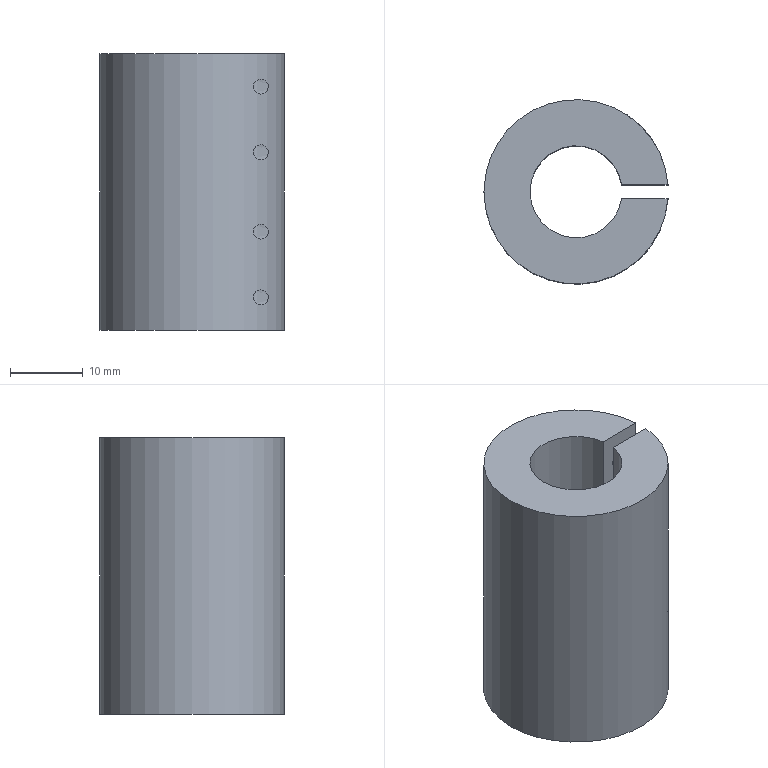Component | NX | BUSHING | 1 solid | 26 faces | volume 13486 mm3 | cylinder 18 | plane 8 | commonest cylinder face diameters 25.4 x5 2.7 x4 5 x4 2.05 x4 12.7 x1